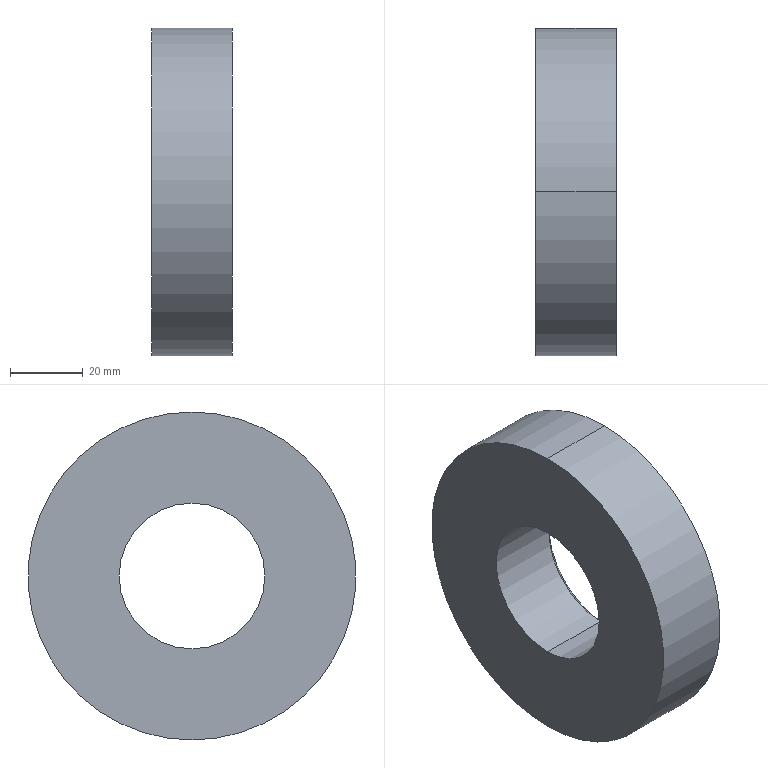Component | SolidWorks | Bearing-1 | 1 solid | 8 faces | box 22 x 90 x 90 mm | volume 112167 mm3 | cylinder 4 | cone 2 | plane 2 | commonest cylinder face diameters 40 x2 90 x2
build123d program:
from build123d import *

# Parameters (mm, degrees)
SKETCH1_R           = 45
SKETCH1_R_2         = 20
BOSS_EXTRUDE1_DEPTH = 22
CHAMFER1_SIZE       = 1.5


with BuildPart() as part:
    # Sketch1 → Boss-Extrude1 (new body)
    with BuildSketch(Plane(origin=(0, 0, 0), x_dir=(0, 0, -1), z_dir=(1, 0, 0))):
        Circle(SKETCH1_R)
        Circle(SKETCH1_R_2, mode=Mode.SUBTRACT)
    extrude(amount=BOSS_EXTRUDE1_DEPTH)

    # Chamfer1
    chamfer1_edges = [part.edges().sort_by_distance(p)[0] for p in [
        (22, 0, 20),
    ]]
    chamfer(chamfer1_edges, length=CHAMFER1_SIZE)


solid = part.part

# Placed as in the assembly
solid = solid.moved(Location((178.528, 15.31, -110), (0, 0, 0)))
STEP:
#1=COLOUR_RGB('',0.7922,0.8196,0.9333);
#2=FILL_AREA_STYLE_COLOUR('',#1);
#3=FILL_AREA_STYLE('',(#2));
#4=SURFACE_STYLE_FILL_AREA(#3);
#5=SURFACE_SIDE_STYLE('',(#4));
#6=SURFACE_STYLE_USAGE(.BOTH.,#5);
#7=PRESENTATION_STYLE_ASSIGNMENT((#6));
#8=CARTESIAN_POINT('',(7.836,0.6028,-3.543));
#9=VERTEX_POINT('',#8);
#10=CARTESIAN_POINT('',(7.836,0.6028,-5.118));
#11=VERTEX_POINT('',#10);
#12=CARTESIAN_POINT('',(7.836,0.6028,-4.331));
#13=DIRECTION('',(1.,0.,0.));
#14=DIRECTION('',(0.,0.,-1.));
#15=AXIS2_PLACEMENT_3D('',#12,#13,#14);
#16=CIRCLE('',#15,0.7874);
#17=EDGE_CURVE('',#9,#11,#16,.T.);
#18=ORIENTED_EDGE('',*,*,#17,.F.);
#19=CARTESIAN_POINT('',(7.895,0.6028,-3.484));
#20=VERTEX_POINT('',#19);
#21=CARTESIAN_POINT('',(7.836,0.6028,-3.543));
#22=DIRECTION('',(0.7071,0.,0.7071));
#23=VECTOR('',#22,39.37);
#24=LINE('',#21,#23);
#25=EDGE_CURVE('',#9,#20,#24,.T.);
#26=ORIENTED_EDGE('',*,*,#25,.T.);
#27=CARTESIAN_POINT('',(7.895,0.6028,-5.177));
#28=VERTEX_POINT('',#27);
#29=CARTESIAN_POINT('',(7.895,0.6028,-4.331));
#30=DIRECTION('',(-1.,0.,0.));
#31=DIRECTION('',(0.,0.,-1.));
#32=AXIS2_PLACEMENT_3D('',#29,#30,#31);
#33=CIRCLE('',#32,0.8465);
#34=EDGE_CURVE('',#28,#20,#33,.T.);
#35=ORIENTED_EDGE('',*,*,#34,.F.);
#36=CARTESIAN_POINT('',(7.836,0.6028,-5.118));
#37=DIRECTION('',(0.7071,0.,-0.7071));
#38=VECTOR('',#37,39.37);
#39=LINE('',#36,#38);
#40=EDGE_CURVE('',#11,#28,#39,.T.);
#41=ORIENTED_EDGE('',*,*,#40,.F.);
#42=EDGE_LOOP('',(#18,#26,#35,#41));
#43=FACE_OUTER_BOUND('',#42,.T.);
#44=CARTESIAN_POINT('',(7.836,0.6028,-4.331));
#45=DIRECTION('',(1.,0.,0.));
#46=DIRECTION('',(0.,0.,-1.));
#47=AXIS2_PLACEMENT_3D('',#44,#45,#46);
#48=CONICAL_SURFACE('',#47,0.7874,0.7854);
#49=ADVANCED_FACE('',(#43),#48,.F.);
#50=ORIENTED_EDGE('',*,*,#17,.T.);
#51=CARTESIAN_POINT('',(7.029,0.6028,-5.118));
#52=VERTEX_POINT('',#51);
#53=CARTESIAN_POINT('',(7.895,0.6028,-5.118));
#54=DIRECTION('',(-1.,0.,0.));
#55=VECTOR('',#54,39.37);
#56=LINE('',#53,#55);
#57=EDGE_CURVE('',#11,#52,#56,.T.);
#58=ORIENTED_EDGE('',*,*,#57,.T.);
#59=CARTESIAN_POINT('',(7.029,0.6028,-3.543));
#60=VERTEX_POINT('',#59);
#61=CARTESIAN_POINT('',(7.029,0.6028,-4.331));
#62=DIRECTION('',(1.,0.,0.));
#63=DIRECTION('',(0.,0.,-1.));
#64=AXIS2_PLACEMENT_3D('',#61,#62,#63);
#65=CIRCLE('',#64,0.7874);
#66=EDGE_CURVE('',#60,#52,#65,.T.);
#67=ORIENTED_EDGE('',*,*,#66,.F.);
#68=CARTESIAN_POINT('',(7.895,0.6028,-3.543));
#69=DIRECTION('',(-1.,0.,0.));
#70=VECTOR('',#69,39.37);
#71=LINE('',#68,#70);
#72=EDGE_CURVE('',#9,#60,#71,.T.);
#73=ORIENTED_EDGE('',*,*,#72,.F.);
#74=EDGE_LOOP('',(#50,#58,#67,#73));
#75=FACE_OUTER_BOUND('',#74,.T.);
#76=CARTESIAN_POINT('',(7.895,0.6028,-4.331));
#77=DIRECTION('',(-1.,0.,0.));
#78=DIRECTION('',(0.,0.,1.));
#79=AXIS2_PLACEMENT_3D('',#76,#77,#78);
#80=CYLINDRICAL_SURFACE('',#79,0.7874);
#81=ADVANCED_FACE('',(#75),#80,.F.);
#82=CARTESIAN_POINT('',(7.895,0.6028,-6.102));
#83=VERTEX_POINT('',#82);
#84=CARTESIAN_POINT('',(7.895,0.6028,-2.559));
#85=VERTEX_POINT('',#84);
#86=CARTESIAN_POINT('',(7.895,0.6028,-4.331));
#87=DIRECTION('',(1.,0.,0.));
#88=DIRECTION('',(0.,0.,-1.));
#89=AXIS2_PLACEMENT_3D('',#86,#87,#88);
#90=CIRCLE('',#89,1.772);
#91=EDGE_CURVE('',#83,#85,#90,.T.);
#92=ORIENTED_EDGE('',*,*,#91,.F.);
#93=CARTESIAN_POINT('',(7.029,0.6028,-6.102));
#94=VERTEX_POINT('',#93);
#95=CARTESIAN_POINT('',(7.895,0.6028,-6.102));
#96=DIRECTION('',(-1.,0.,0.));
#97=VECTOR('',#96,39.37);
#98=LINE('',#95,#97);
#99=EDGE_CURVE('',#83,#94,#98,.T.);
#100=ORIENTED_EDGE('',*,*,#99,.T.);
#101=CARTESIAN_POINT('',(7.029,0.6028,-2.559));
#102=VERTEX_POINT('',#101);
#103=CARTESIAN_POINT('',(7.029,0.6028,-4.331));
#104=DIRECTION('',(1.,0.,0.));
#105=DIRECTION('',(0.,0.,-1.));
#106=AXIS2_PLACEMENT_3D('',#103,#104,#105);
#107=CIRCLE('',#106,1.772);
#108=EDGE_CURVE('',#94,#102,#107,.T.);
#109=ORIENTED_EDGE('',*,*,#108,.T.);
#110=CARTESIAN_POINT('',(7.895,0.6028,-2.559));
#111=DIRECTION('',(-1.,0.,0.));
#112=VECTOR('',#111,39.37);
#113=LINE('',#110,#112);
#114=EDGE_CURVE('',#85,#102,#113,.T.);
#115=ORIENTED_EDGE('',*,*,#114,.F.);
#116=EDGE_LOOP('',(#92,#100,#109,#115));
#117=FACE_OUTER_BOUND('',#116,.T.);
#118=CARTESIAN_POINT('',(7.895,0.6028,-4.331));
#119=DIRECTION('',(-1.,0.,0.));
#120=DIRECTION('',(0.,0.,1.));
#121=AXIS2_PLACEMENT_3D('',#118,#119,#120);
#122=CYLINDRICAL_SURFACE('',#121,1.772);
#123=ADVANCED_FACE('',(#117),#122,.T.);
#124=ORIENTED_EDGE('',*,*,#34,.T.);
#125=CARTESIAN_POINT('',(7.895,0.6028,-4.331));
#126=DIRECTION('',(-1.,0.,0.));
#127=DIRECTION('',(0.,0.,-1.));
#128=AXIS2_PLACEMENT_3D('',#125,#126,#127);
#129=CIRCLE('',#128,0.8465);
#130=EDGE_CURVE('',#20,#28,#129,.T.);
#131=ORIENTED_EDGE('',*,*,#130,.T.);
#132=EDGE_LOOP('',(#124,#131));
#133=FACE_BOUND('',#132,.T.);
#134=CARTESIAN_POINT('',(7.895,0.6028,-4.331));
#135=DIRECTION('',(1.,0.,0.));
#136=DIRECTION('',(0.,0.,-1.));
#137=AXIS2_PLACEMENT_3D('',#134,#135,#136);
#138=CIRCLE('',#137,1.772);
#139=EDGE_CURVE('',#85,#83,#138,.T.);
#140=ORIENTED_EDGE('',*,*,#139,.T.);
#141=ORIENTED_EDGE('',*,*,#91,.T.);
#142=EDGE_LOOP('',(#140,#141));
#143=FACE_OUTER_BOUND('',#142,.T.);
#144=CARTESIAN_POINT('',(7.895,0.6028,-4.331));
#145=DIRECTION('',(1.,0.,0.));
#146=DIRECTION('',(0.,0.,-1.));
#147=AXIS2_PLACEMENT_3D('',#144,#145,#146);
#148=PLANE('',#147);
#149=ADVANCED_FACE('',(#133,#143),#148,.T.);
#150=CARTESIAN_POINT('',(7.029,0.6028,-4.331));
#151=DIRECTION('',(1.,0.,0.));
#152=DIRECTION('',(0.,0.,-1.));
#153=AXIS2_PLACEMENT_3D('',#150,#151,#152);
#154=CIRCLE('',#153,1.772);
#155=EDGE_CURVE('',#102,#94,#154,.T.);
#156=ORIENTED_EDGE('',*,*,#155,.F.);
#157=ORIENTED_EDGE('',*,*,#108,.F.);
#158=EDGE_LOOP('',(#156,#157));
#159=FACE_OUTER_BOUND('',#158,.T.);
#160=ORIENTED_EDGE('',*,*,#66,.T.);
#161=CARTESIAN_POINT('',(7.029,0.6028,-4.331));
#162=DIRECTION('',(1.,0.,0.));
#163=DIRECTION('',(0.,0.,-1.));
#164=AXIS2_PLACEMENT_3D('',#161,#162,#163);
#165=CIRCLE('',#164,0.7874);
#166=EDGE_CURVE('',#52,#60,#165,.T.);
#167=ORIENTED_EDGE('',*,*,#166,.T.);
#168=EDGE_LOOP('',(#160,#167));
#169=FACE_BOUND('',#168,.T.);
#170=CARTESIAN_POINT('',(7.029,0.6028,-4.331));
#171=DIRECTION('',(1.,0.,0.));
#172=DIRECTION('',(0.,0.,-1.));
#173=AXIS2_PLACEMENT_3D('',#170,#171,#172);
#174=PLANE('',#173);
#175=ADVANCED_FACE('',(#159,#169),#174,.F.);
#176=ORIENTED_EDGE('',*,*,#99,.F.);
#177=ORIENTED_EDGE('',*,*,#139,.F.);
#178=ORIENTED_EDGE('',*,*,#114,.T.);
#179=ORIENTED_EDGE('',*,*,#155,.T.);
#180=EDGE_LOOP('',(#176,#177,#178,#179));
#181=FACE_OUTER_BOUND('',#180,.T.);
#182=CARTESIAN_POINT('',(7.895,0.6028,-4.331));
#183=DIRECTION('',(-1.,0.,0.));
#184=DIRECTION('',(0.,0.,1.));
#185=AXIS2_PLACEMENT_3D('',#182,#183,#184);
#186=CYLINDRICAL_SURFACE('',#185,1.772);
#187=ADVANCED_FACE('',(#181),#186,.T.);
#188=ORIENTED_EDGE('',*,*,#57,.F.);
#189=CARTESIAN_POINT('',(7.836,0.6028,-4.331));
#190=DIRECTION('',(1.,0.,0.));
#191=DIRECTION('',(0.,0.,-1.));
#192=AXIS2_PLACEMENT_3D('',#189,#190,#191);
#193=CIRCLE('',#192,0.7874);
#194=EDGE_CURVE('',#11,#9,#193,.T.);
#195=ORIENTED_EDGE('',*,*,#194,.T.);
#196=ORIENTED_EDGE('',*,*,#72,.T.);
#197=ORIENTED_EDGE('',*,*,#166,.F.);
#198=EDGE_LOOP('',(#188,#195,#196,#197));
#199=FACE_OUTER_BOUND('',#198,.T.);
#200=CARTESIAN_POINT('',(7.895,0.6028,-4.331));
#201=DIRECTION('',(-1.,0.,0.));
#202=DIRECTION('',(0.,0.,1.));
#203=AXIS2_PLACEMENT_3D('',#200,#201,#202);
#204=CYLINDRICAL_SURFACE('',#203,0.7874);
#205=ADVANCED_FACE('',(#199),#204,.F.);
#206=ORIENTED_EDGE('',*,*,#25,.F.);
#207=ORIENTED_EDGE('',*,*,#194,.F.);
#208=ORIENTED_EDGE('',*,*,#40,.T.);
#209=ORIENTED_EDGE('',*,*,#130,.F.);
#210=EDGE_LOOP('',(#206,#207,#208,#209));
#211=FACE_OUTER_BOUND('',#210,.T.);
#212=CARTESIAN_POINT('',(7.836,0.6028,-4.331));
#213=DIRECTION('',(1.,0.,0.));
#214=DIRECTION('',(0.,0.,-1.));
#215=AXIS2_PLACEMENT_3D('',#212,#213,#214);
#216=CONICAL_SURFACE('',#215,0.7874,0.7854);
#217=ADVANCED_FACE('',(#211),#216,.F.);
#218=CLOSED_SHELL('',(#49,#81,#123,#149,#175,#187,#205,#217));
#219=MANIFOLD_SOLID_BREP('',#218);
#220=STYLED_ITEM('',(#7),#219);
#221=PRESENTATION_LAYER_ASSIGNMENT('','',(#220));
#222=(LENGTH_UNIT()NAMED_UNIT(*)SI_UNIT($,.METRE.));
#223=LENGTH_MEASURE_WITH_UNIT(LENGTH_MEASURE(0.0254),#222);
#224=DIMENSIONAL_EXPONENTS(1.,0.,0.,0.,0.,0.,0.);
#225=(CONVERSION_BASED_UNIT('',#223)LENGTH_UNIT()NAMED_UNIT(#224));
#226=UNCERTAINTY_MEASURE_WITH_UNIT(LENGTH_MEASURE(0.00001),#225,'','');
#227=(NAMED_UNIT(*)PLANE_ANGLE_UNIT()SI_UNIT($,.RADIAN.));
#228=(NAMED_UNIT(*)SI_UNIT($,.STERADIAN.)SOLID_ANGLE_UNIT());
#229=(GEOMETRIC_REPRESENTATION_CONTEXT(3)GLOBAL_UNCERTAINTY_ASSIGNED_CONTEXT((#226))GLOBAL_UNIT_ASSIGNED_CONTEXT((#225,#227,#228))REPRESENTATION_CONTEXT('',''));
#230=MECHANICAL_DESIGN_GEOMETRIC_PRESENTATION_REPRESENTATION('',(#220),#229);
#231=CARTESIAN_POINT('',(0.,0.,0.));
#232=DIRECTION('',(0.,0.,1.));
#233=DIRECTION('',(1.,0.,0.));
#234=AXIS2_PLACEMENT_3D('',#231,#232,#233);
#235=(LENGTH_UNIT()NAMED_UNIT(*)SI_UNIT($,.METRE.));
#236=LENGTH_MEASURE_WITH_UNIT(LENGTH_MEASURE(0.0254),#235);
#237=DIMENSIONAL_EXPONENTS(1.,0.,0.,0.,0.,0.,0.);
#238=(CONVERSION_BASED_UNIT('',#236)LENGTH_UNIT()NAMED_UNIT(#237));
#239=UNCERTAINTY_MEASURE_WITH_UNIT(LENGTH_MEASURE(0.00001),#238,'','');
#240=(NAMED_UNIT(*)PLANE_ANGLE_UNIT()SI_UNIT($,.RADIAN.));
#241=(NAMED_UNIT(*)SI_UNIT($,.STERADIAN.)SOLID_ANGLE_UNIT());
#242=(GEOMETRIC_REPRESENTATION_CONTEXT(3)GLOBAL_UNCERTAINTY_ASSIGNED_CONTEXT((#239))GLOBAL_UNIT_ASSIGNED_CONTEXT((#238,#240,#241))REPRESENTATION_CONTEXT('',''));
#243=ADVANCED_BREP_SHAPE_REPRESENTATION('',(#219,#234),#242);